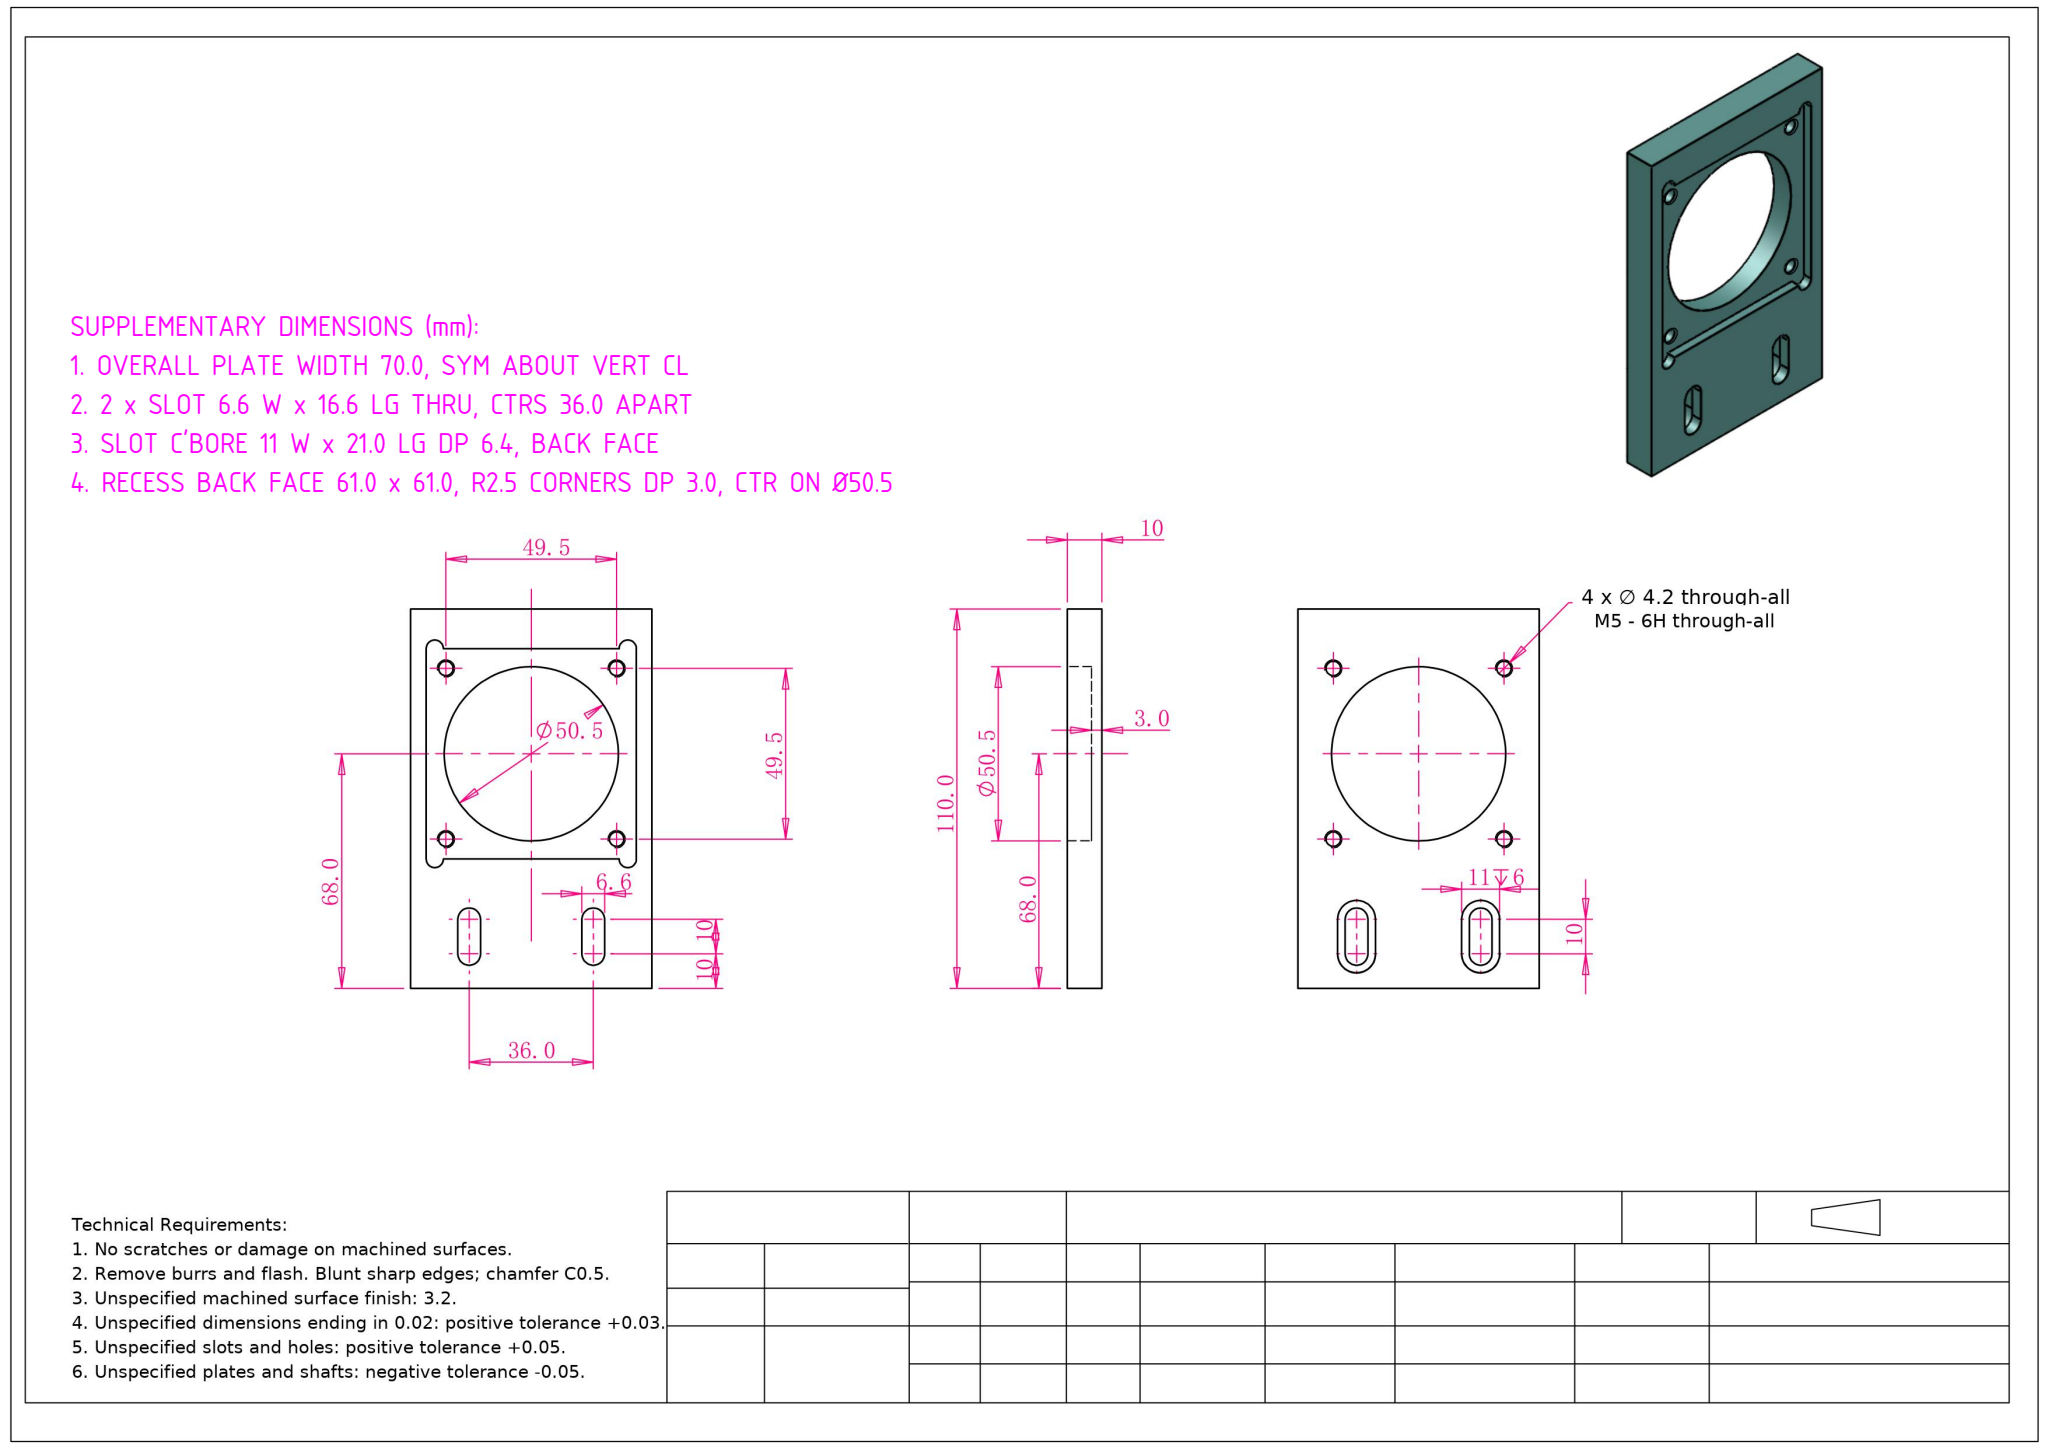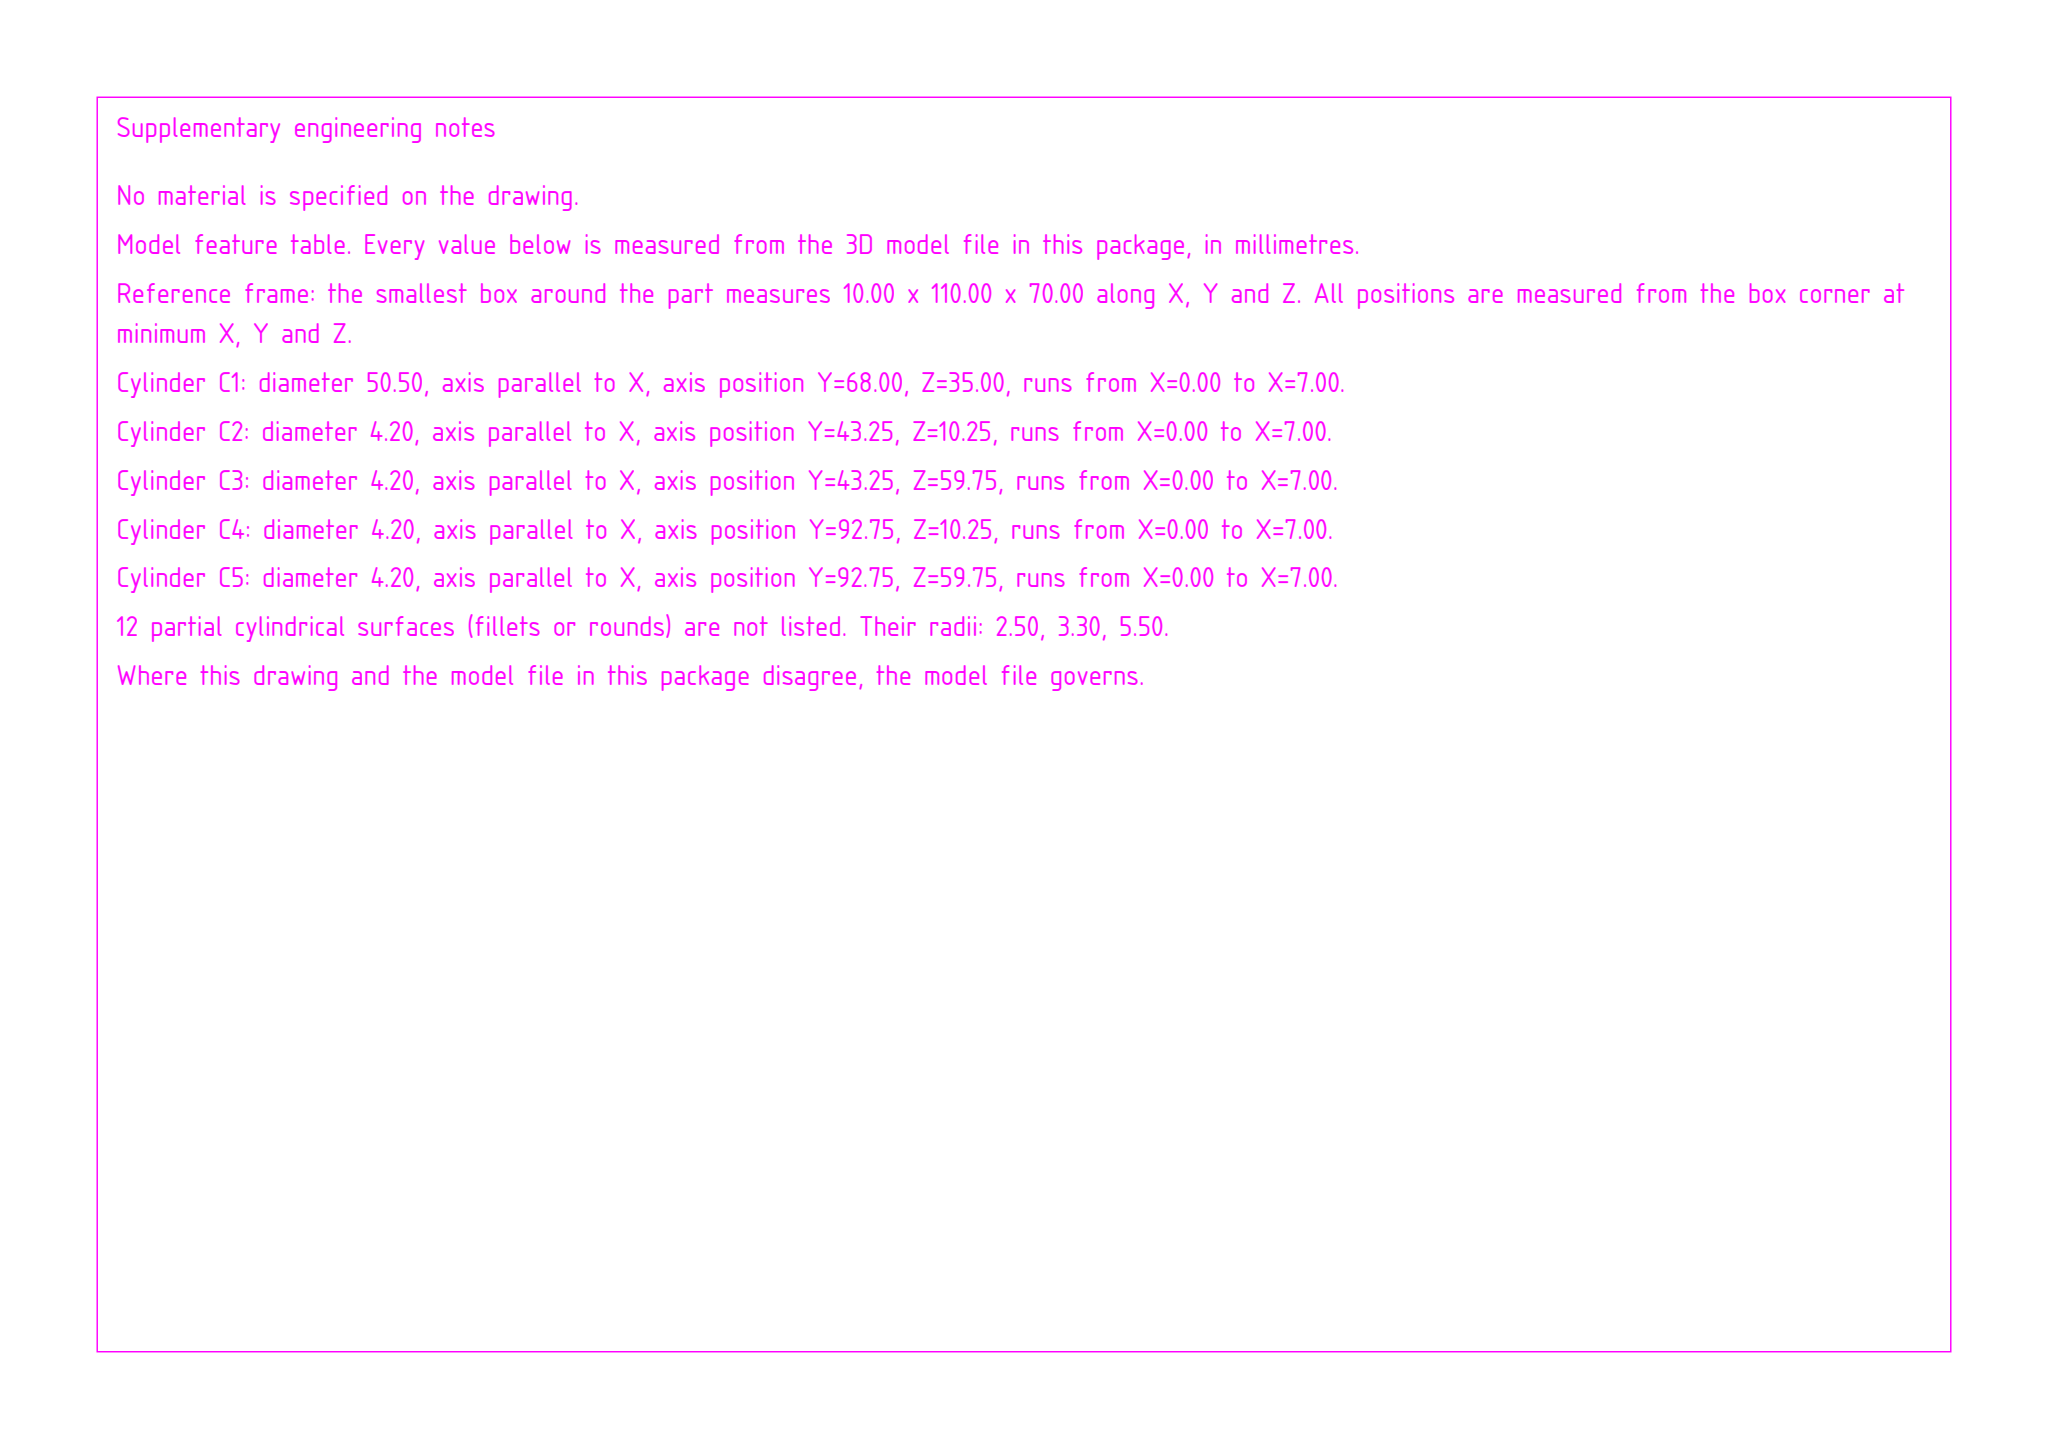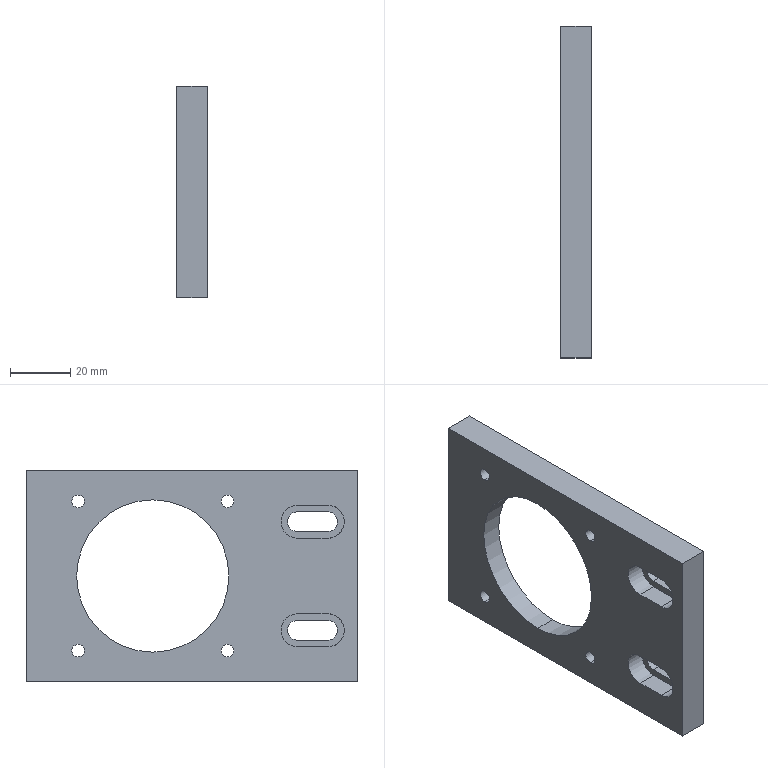Part | SolidWorks | mm | 1 solid | 49 faces | box 10 x 110 x 70 mm | volume 47965 mm3 | cylinder 22 | plane 21 | cone 6 | commonest cylinder face diameters 4.2 x8 6.6 x4 11 x4 5 x4 50.5 x2
build123d program:
from build123d import *

# Parameters (mm, degrees)
EXTRUDE_THIN1_DEPTH                            = 35
SKETCH2_R                                      = 25.25
CUT_EXTRUDE1_DEPTH                             = 123.168
CUT_EXTRUDE2_DEPTH                             = 10
M5_TAPPED_HOLE1_D                              = 4.2
SKETCH9_W                                      = 40
SKETCH9_H                                      = 10
CUT_EXTRUDE4_DEPTH                             = 140.642
M6_HEX_SOCKET_HEAD_CAP_SCREW_CBORE1_AT_2_COUNT = 2
M6_HEX_SOCKET_HEAD_CAP_SCREW_CBORE1_AT_2_PITCH = 36
CUT_EXTRUDE5_DEPTH                             = 6.4
CUT_EXTRUDE6_DEPTH                             = 116.611
SKETCH16_W                                     = 61
SKETCH16_H                                     = 61
CUT_EXTRUDE7_DEPTH                             = 3
SKETCH18_R                                     = 2.5
CUT_EXTRUDE9_DEPTH                             = 3


with BuildPart() as part:
    # Sketch1 → Extrude-Thin1 (new, symmetric)
    with BuildSketch(Plane.XY):
        Polygon((0, 110), (0, 0), (50, 0), (50, 10), (10, 10), (10, 110), align=None)
    extrude(amount=EXTRUDE_THIN1_DEPTH, both=True)

    # Sketch2 → Cut-Extrude1 (cut, through all)
    with BuildSketch(Plane(origin=(10, 0, 0), x_dir=(0, 0, -1), z_dir=(1, 0, 0))):
        with Locations((0, 68)):
            Circle(SKETCH2_R)
    extrude(amount=-CUT_EXTRUDE1_DEPTH, mode=Mode.SUBTRACT)

    # Sketch3 → Cut-Extrude2 (cut)
    with BuildSketch(Plane(origin=(0, 10, 0), x_dir=(1, 0, 0), z_dir=(0, 1, 0))):
        with BuildLine():
            Line((19, 19.5), (25, 19.5))
            ThreePointArc((25, 19.5), (29.5, 15), (25, 10.5))
            Line((25, 10.5), (19, 10.5))
            ThreePointArc((19, 10.5), (14.5, 15), (19, 19.5))
        make_face()
        with BuildLine():
            Line((37, 19.5), (43, 19.5))
            ThreePointArc((43, 19.5), (47.5, 15), (43, 10.5))
            Line((43, 10.5), (37, 10.5))
            ThreePointArc((37, 10.5), (32.5, 15), (37, 19.5))
        make_face()
        with BuildLine():
            Line((37, -19.5), (43, -19.5))
            ThreePointArc((43, -19.5), (47.5, -15), (43, -10.5))
            Line((43, -10.5), (37, -10.5))
            ThreePointArc((37, -10.5), (32.5, -15), (37, -19.5))
        make_face()
        with BuildLine():
            Line((19, -19.5), (25, -19.5))
            ThreePointArc((25, -19.5), (29.5, -15), (25, -10.5))
            Line((25, -10.5), (19, -10.5))
            ThreePointArc((19, -10.5), (14.5, -15), (19, -19.5))
        make_face()
    extrude(amount=-CUT_EXTRUDE2_DEPTH, mode=Mode.SUBTRACT)

    # M5 Tapped Hole1 (through all)
    with Locations(Plane(origin=(10, 0, 0), x_dir=(0, 0, -1), z_dir=(1, 0, 0))):
        with Locations((-24.749, 92.749), (24.749, 92.749), (24.749, 43.251), (-24.749, 43.251)):
            Hole(M5_TAPPED_HOLE1_D / 2)

    # Sketch9 → Cut-Extrude4 (cut, through all)
    with BuildSketch(Plane.XY.offset(35)):
        with Locations((30, 5)):
            Rectangle(SKETCH9_W, SKETCH9_H)
    extrude(amount=-CUT_EXTRUDE4_DEPTH, mode=Mode.SUBTRACT)

    # Sketch13 → M6 Hex Socket Head Cap Screw CBORE1 (revolve, cut)
    with BuildSketch(Plane(origin=(0, 10, 18), x_dir=(0, 0, 1), z_dir=(0, 1, 0))):
        Polygon((0, 0), (0, 10), (3.3, 10), (3.3, 6.4), (5.5, 6.4), (5.5, 0.025), (5.525, 0), align=None)
    m6_hex_socket_head_cap_screw_cbore1 = revolve(axis=Axis((-6.35, 10, 18), (1, 0, 0)), mode=Mode.SUBTRACT)

    # M6 Hex Socket Head Cap Screw CBORE1 at 2: M6 Hex Socket Head Cap Screw CBORE1 ×2
    with Locations(*[(0, 0, -i * M6_HEX_SOCKET_HEAD_CAP_SCREW_CBORE1_AT_2_PITCH) for i in range(1, M6_HEX_SOCKET_HEAD_CAP_SCREW_CBORE1_AT_2_COUNT)]):
        add(m6_hex_socket_head_cap_screw_cbore1, mode=Mode.SUBTRACT)

    # Sketch14 → Cut-Extrude5 (cut)
    with BuildSketch(Plane.ZY):
        with BuildLine():
            Line((-12.5, 20), (-12.5, 10))
            ThreePointArc((-12.5, 10), (-18, 4.5), (-23.5, 10))
            Line((-23.5, 10), (-23.5, 20))
            ThreePointArc((-23.5, 20), (-18, 25.5), (-12.5, 20))
        make_face()
        with BuildLine():
            Line((12.5, 20), (12.5, 10))
            ThreePointArc((12.5, 10), (18, 4.5), (23.5, 10))
            Line((23.5, 10), (23.5, 20))
            ThreePointArc((23.5, 20), (18, 25.5), (12.5, 20))
        make_face()
    extrude(amount=-CUT_EXTRUDE5_DEPTH, mode=Mode.SUBTRACT)

    # Sketch15 → Cut-Extrude6 (cut, through all)
    with BuildSketch(Plane.ZY.offset(-6.4)):
        with BuildLine():
            Line((-21.3, 10), (-21.3, 20))
            ThreePointArc((-21.3, 20), (-18, 23.3), (-14.7, 20))
            Line((-14.7, 20), (-14.7, 10))
            ThreePointArc((-14.7, 10), (-18, 6.7), (-21.3, 10))
        make_face()
        with BuildLine():
            Line((21.3, 10), (21.3, 20))
            ThreePointArc((21.3, 20), (18, 23.3), (14.7, 20))
            Line((14.7, 20), (14.7, 10))
            ThreePointArc((14.7, 10), (18, 6.7), (21.3, 10))
        make_face()
    extrude(amount=-CUT_EXTRUDE6_DEPTH, mode=Mode.SUBTRACT)

    # Sketch16 → Cut-Extrude7 (cut)
    with BuildSketch(Plane(origin=(10, 0, 0), x_dir=(0, 0, -1), z_dir=(1, 0, 0))):
        with Locations((0, 68)):
            Rectangle(SKETCH16_W, SKETCH16_H)
    extrude(amount=-CUT_EXTRUDE7_DEPTH, mode=Mode.SUBTRACT)

    # Sketch18 → Cut-Extrude9 (cut)
    with BuildSketch(Plane(origin=(10, 0, 0), x_dir=(0, 0, -1), z_dir=(1, 0, 0))):
        with Locations((-28, 98.5)):
            Circle(SKETCH18_R)
        with Locations((28, 98.5)):
            Circle(SKETCH18_R)
        with Locations((-28, 37.5)):
            Circle(SKETCH18_R)
        with Locations((28, 37.5)):
            Circle(SKETCH18_R)
    extrude(amount=-CUT_EXTRUDE9_DEPTH, mode=Mode.SUBTRACT)


solid = part.part